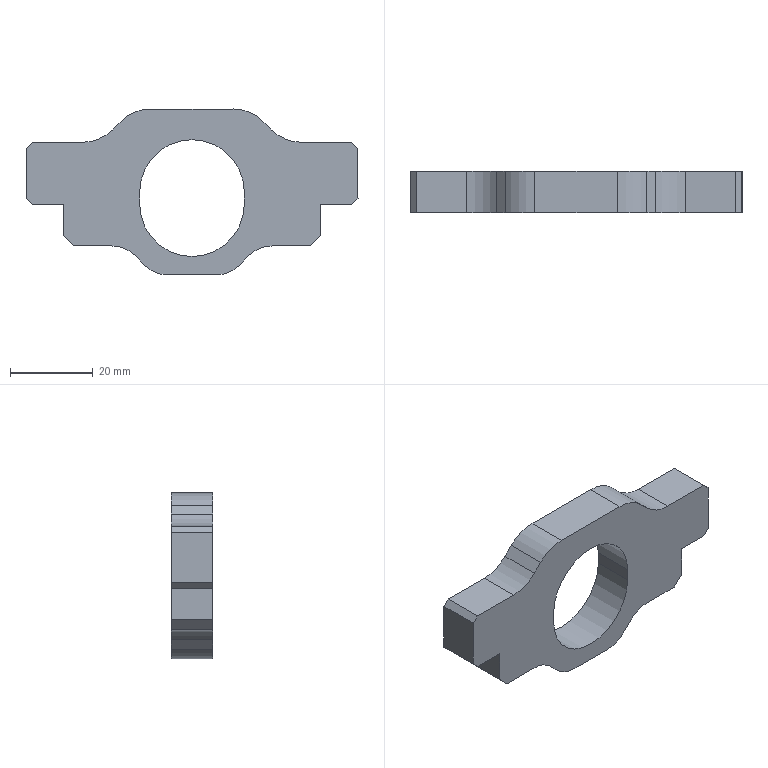Component | NX | MODEL20 | 1 solid | 38 faces | volume 17007 mm3 | plane 28 | cylinder 10 | commonest cylinder face diameters 20 x4 16 x4 25.2 x2